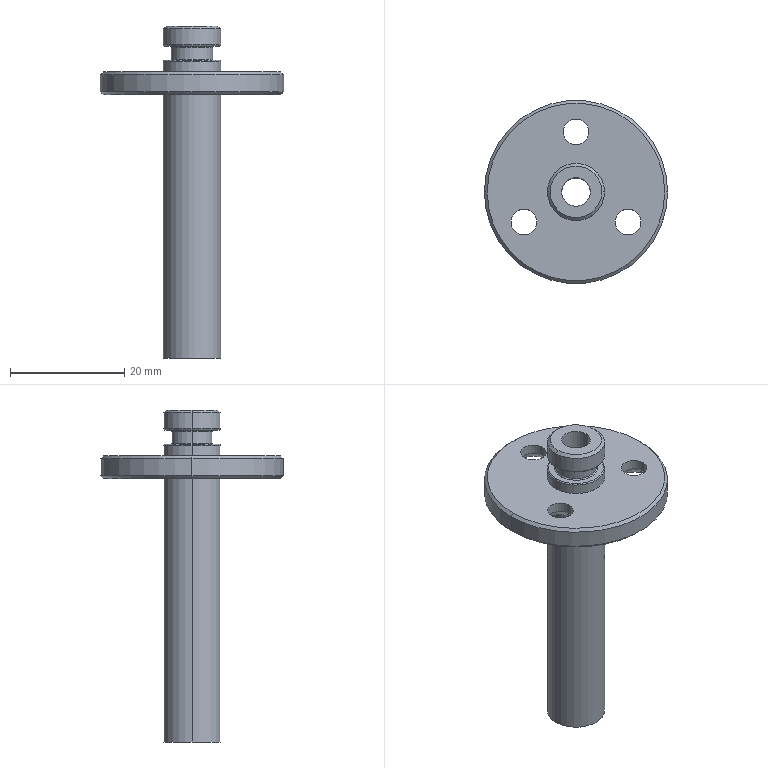Component | SolidWorks | 6.11-1937032104-0-1 | 1 solid | 44 faces | box 32 x 32 x 58 mm | volume 5865 mm3 | cylinder 18 | cone 12 | torus 8 | plane 6 | commonest cylinder face diameters 10 x6 4.5 x6 5 x2 7.2 x2 32 x2 | material Cr12MoV
build123d program:
from build123d import *

# Parameters (mm, degrees)
SKETCH1_R                                    = 5
BOSS_EXTRUDE1_DEPTH                          = 50
SKETCH2_R                                    = 16
BOSS_EXTRUDE2_DEPTH                          = 4
M4_HEXAGON_SOCKET_COUNTERSUNK_HEAD_S_2_COUNT = 2
M4_HEXAGON_SOCKET_COUNTERSUNK_HEAD_S_2_PITCH = 18.187
M4_HEXAGON_SOCKET_COUNTERSUNK_HEAD_S_3_COUNT = 2
M4_HEXAGON_SOCKET_COUNTERSUNK_HEAD_S_3_PITCH = 18.187
BOSS_EXTRUDE3_START                          = 8
SKETCH6_R                                    = 5
BOSS_EXTRUDE3_DEPTH                          = 8
CUT_EXTRUDE_THIN1_START                      = 4.5
SKETCH7_R                                    = 5
SKETCH7_R_2                                  = 3.6
CUT_EXTRUDE_THIN1_DEPTH                      = 2.5
M6_TAPPED_HOLE1_D                            = 5
CHAMFER1_SIZE                                = 0.5
FILLET1_R                                    = 0.2


with BuildPart() as part:
    # Sketch1 → Boss-Extrude1 (new body)
    with BuildSketch(Plane.XY):
        Circle(SKETCH1_R)
    extrude(amount=BOSS_EXTRUDE1_DEPTH)

    # Sketch2 → Boss-Extrude2 (add)
    with BuildSketch(Plane(origin=(0, 0, 0), x_dir=(-1, 0, 0), z_dir=(0, 0, -1))):
        Circle(SKETCH2_R)
    extrude(amount=-BOSS_EXTRUDE2_DEPTH)

    # Sketch3 → M4 Hexagon Socket Countersunk Head Screw (revolve, cut)
    with BuildSketch(Plane(origin=(0, 10.5, 4), x_dir=(0, -1, 0), z_dir=(1, 0, 0))):
        Polygon((0, 0), (0, 4), (2.25, 4), (2.25, 2.23), (4.48, 0), align=None)
    m4_hexagon_socket_countersunk_head_screw = revolve(axis=Axis((0, 10.5, 10.35), (0, 0, -1)), mode=Mode.SUBTRACT)

    # M4 Hexagon Socket Countersunk Head S 2: M4 Hexagon Socket Countersunk Head Screw ×2
    with Locations(*[Vector(-0.5, -0.866, 0) * (i * M4_HEXAGON_SOCKET_COUNTERSUNK_HEAD_S_2_PITCH) for i in range(1, M4_HEXAGON_SOCKET_COUNTERSUNK_HEAD_S_2_COUNT)]):
        add(m4_hexagon_socket_countersunk_head_screw, mode=Mode.SUBTRACT)

    # M4 Hexagon Socket Countersunk Head S 3: M4 Hexagon Socket Countersunk Head Screw ×2
    with Locations(*[Vector(0.5, -0.866, 0) * (i * M4_HEXAGON_SOCKET_COUNTERSUNK_HEAD_S_3_PITCH) for i in range(1, M4_HEXAGON_SOCKET_COUNTERSUNK_HEAD_S_3_COUNT)]):
        add(m4_hexagon_socket_countersunk_head_screw, mode=Mode.SUBTRACT)

    # Sketch6 → Boss-Extrude3 (add)
    with BuildSketch(Plane(origin=(0, 0, 0), x_dir=(-1, 0, 0), z_dir=(0, 0, -1)).offset(BOSS_EXTRUDE3_START)):
        Circle(SKETCH6_R)
    extrude(amount=-BOSS_EXTRUDE3_DEPTH)

    # Sketch7 → Cut-Extrude-Thin1 (cut)
    with BuildSketch(Plane(origin=(0, 0, 0), x_dir=(-1, 0, 0), z_dir=(0, 0, -1)).offset(CUT_EXTRUDE_THIN1_START)):
        Circle(SKETCH7_R)
        Circle(SKETCH7_R_2, mode=Mode.SUBTRACT)
    extrude(amount=-CUT_EXTRUDE_THIN1_DEPTH, mode=Mode.SUBTRACT)

    # M6 Tapped Hole1 (through all)
    with Locations(Plane.XY.offset(50)):
        with Locations((0, 0)):
            Hole(M6_TAPPED_HOLE1_D / 2)

    # Chamfer1
    chamfer1_edges = [part.edges().sort_by_distance(p)[0] for p in [
        (5, 0, -8),
        (16, 0, 0),
        (16, 0, 4),
    ]]
    chamfer(chamfer1_edges, length=CHAMFER1_SIZE)

    # Fillet1
    fillet1_edges = [part.edges().sort_by_distance(p)[0] for p in [
        (5, 0, -4.5),
        (3.6, 0, -2),
        (5, 0, -2),
        (3.6, 0, -4.5),
    ]]
    fillet(fillet1_edges, radius=FILLET1_R)


solid = part.part

# Placed as in the assembly
solid = solid.moved(Location((0, 45, 4), (-180, 0, 180)))